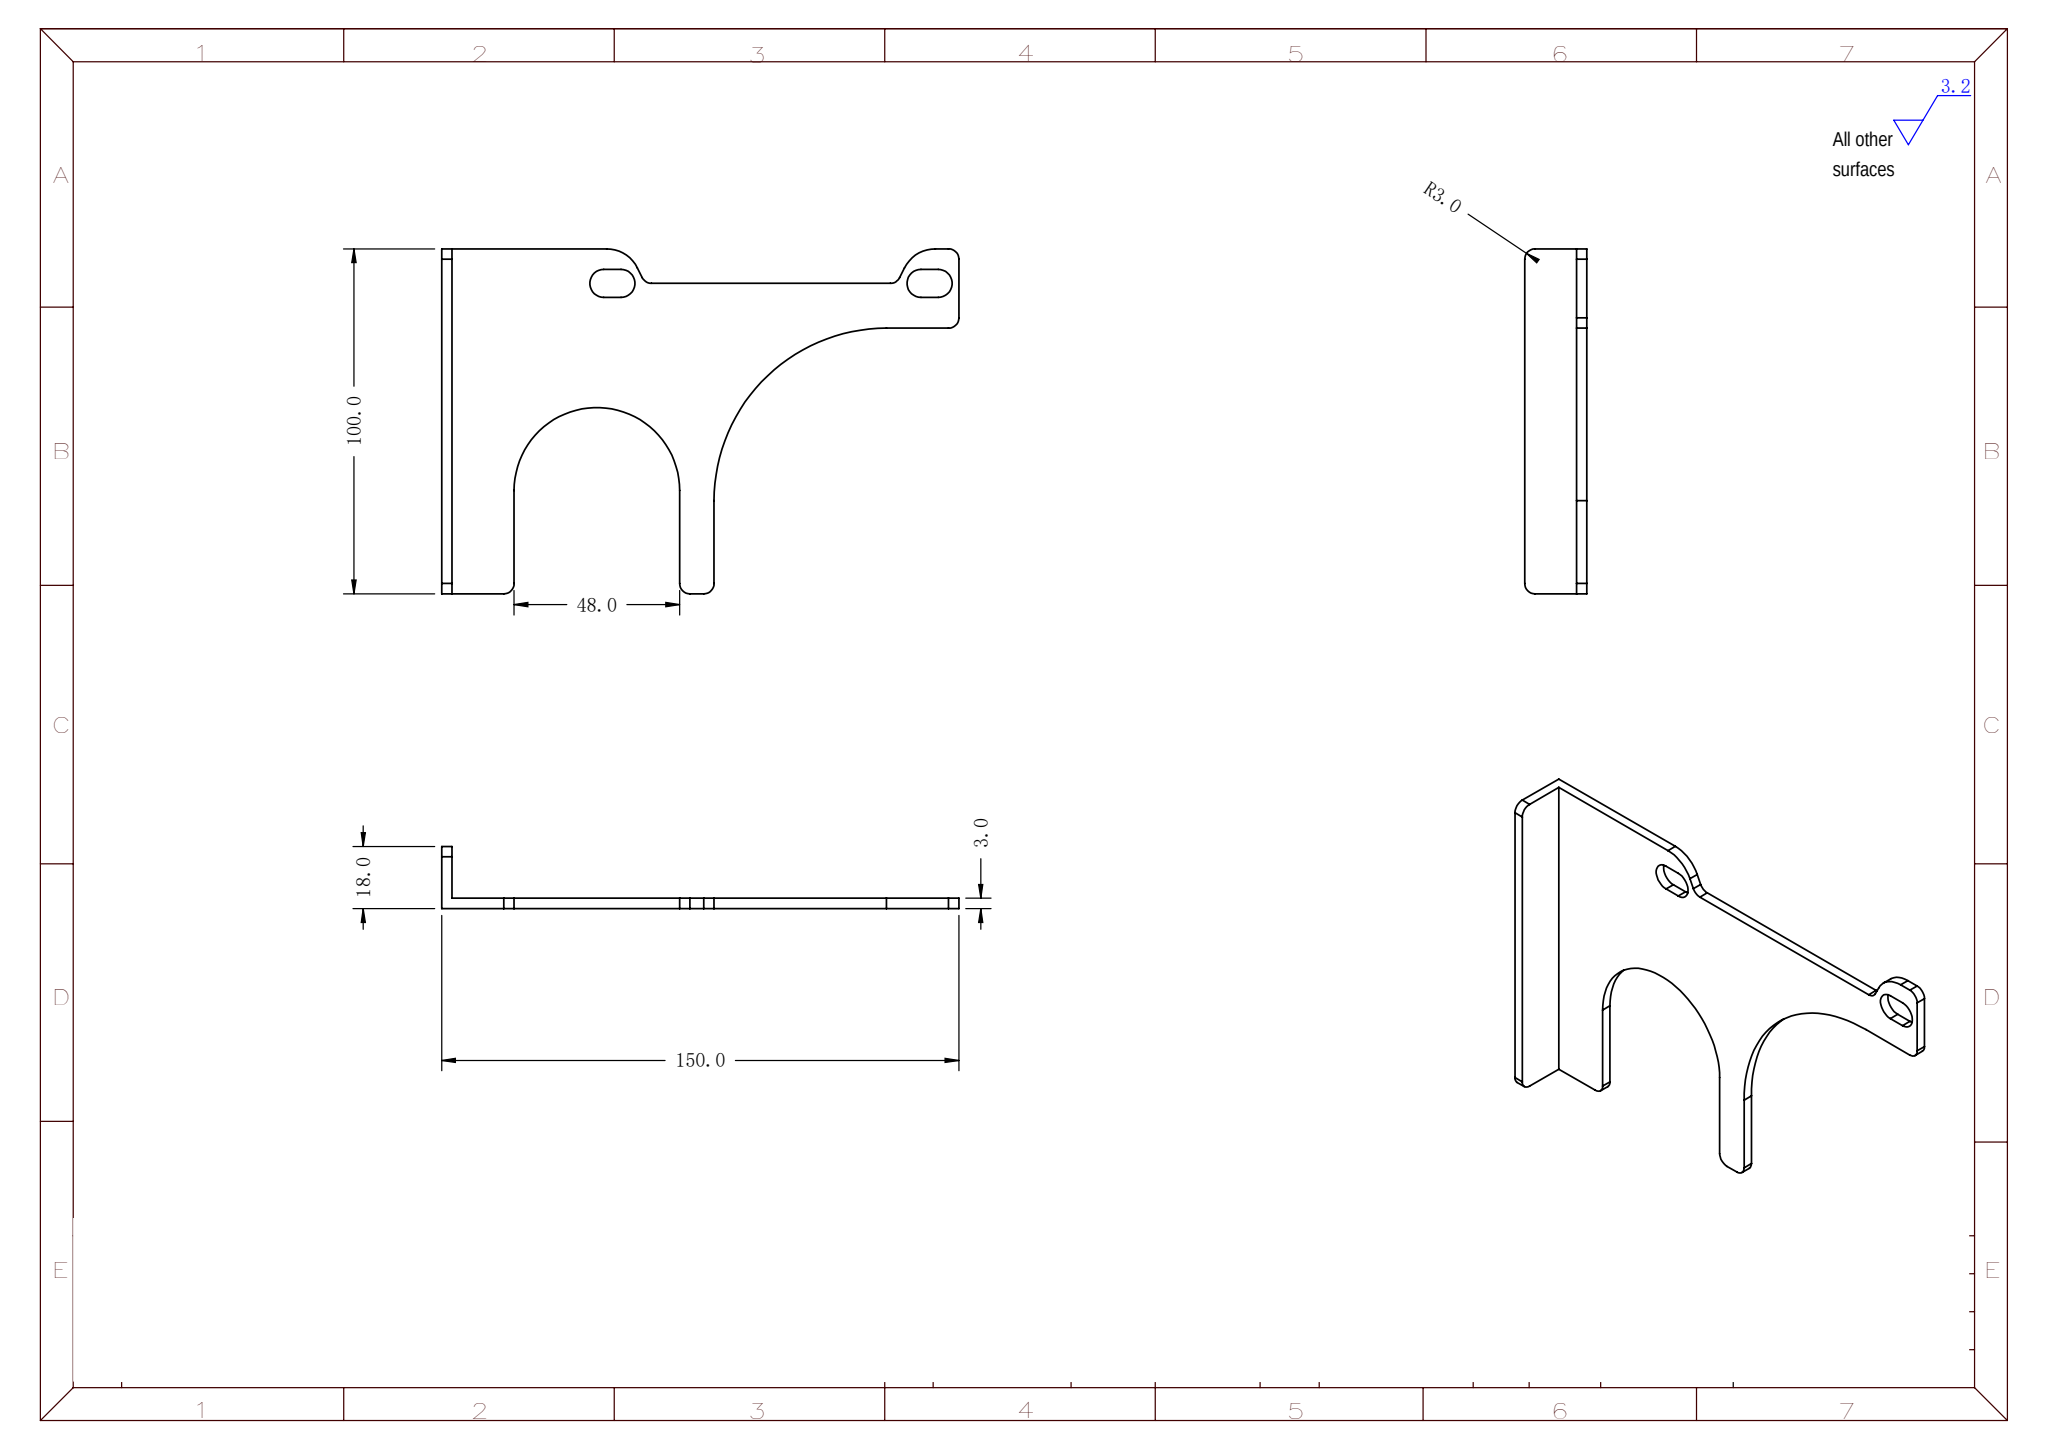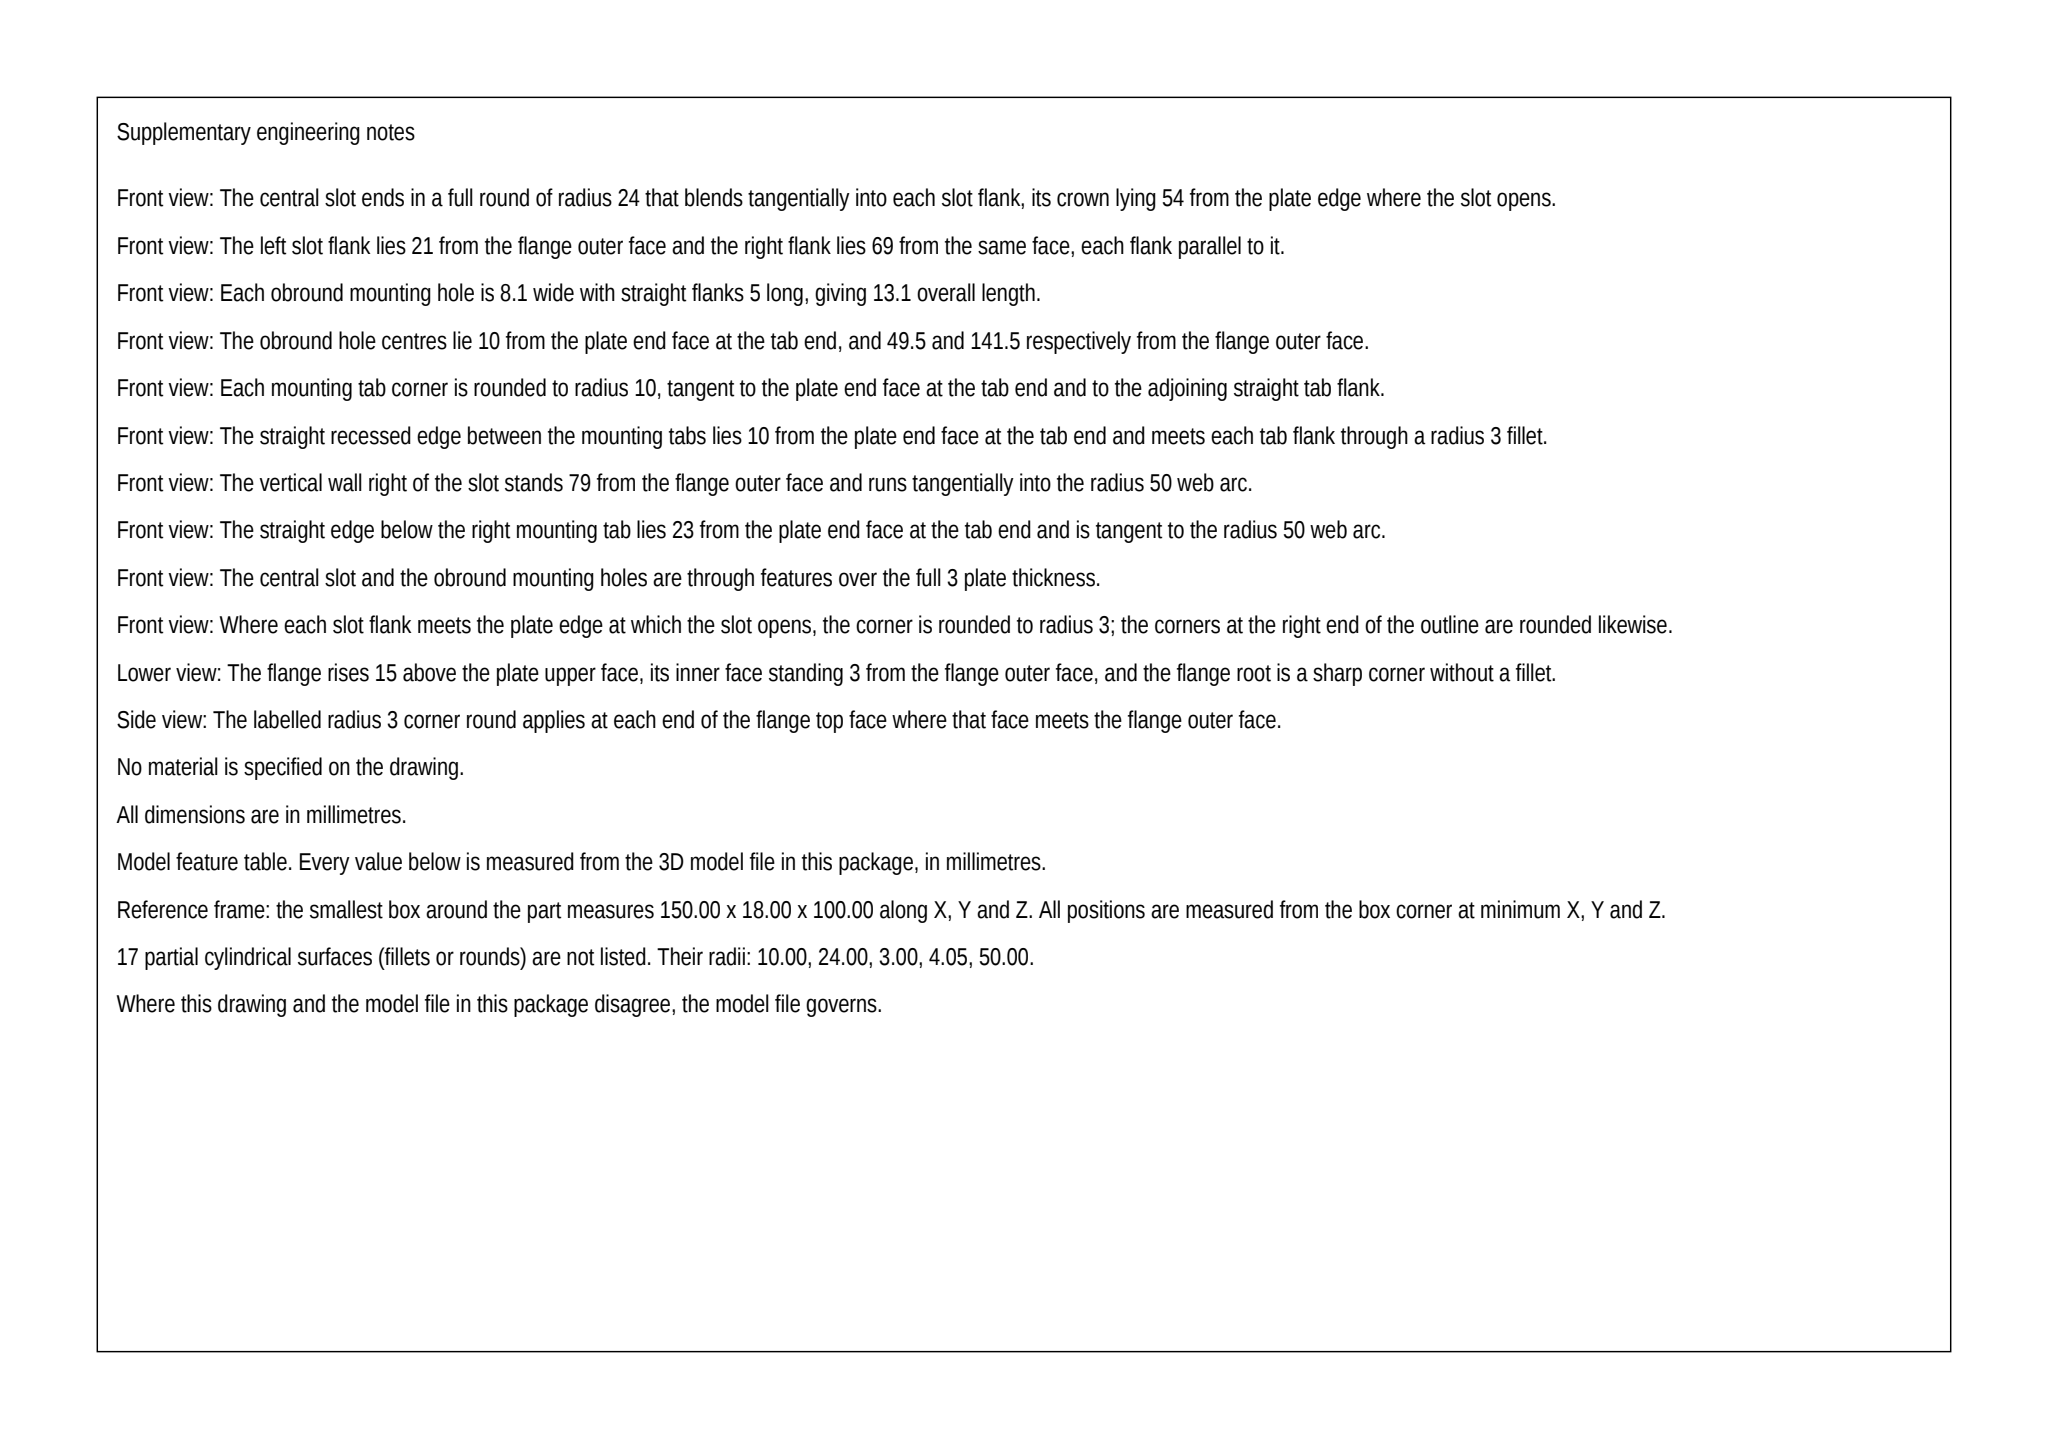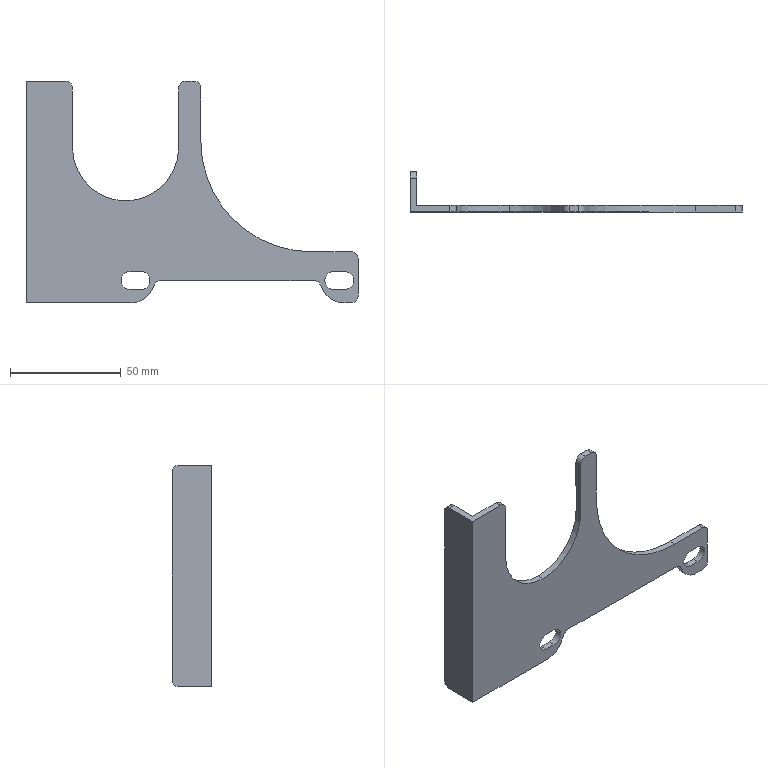Part | SolidWorks | mm | 1 solid | 39 faces | box 150 x 18 x 100 mm | volume 24706 mm3 | plane 21 | cylinder 18 | commonest cylinder face diameters 6 x9 8.1 x4 48 x2 20 x2 100 x1
Drawing notes:
ALL DIMENSIONS IN MILLIMETRES (mm). | from the solid: STEP bbox_xyz [150.0,18.0,100.0] given in mm
2X SLOT 8.1 WIDE X 13.1 LONG THRU (3.0 PLATE); SLOT CENTRES AT X=49.5 AND X=141.5 FROM LEFT EDGE (X0), BOTH 10.0 BELOW TOP EDGE. CENTRE-TO-CENTRE 92.0. | from the solid: cylinders dia 8.1 axis y at x=47.0 & 52.0 and x=139.0 & 144.0, all z=10.0, length 3.0
2X R10.0 LUG OUTER ARC: ARC CENTRES AT X=47.82 AND X=143.18 FROM LEFT EDGE (X0), 10.0 BELOW TOP EDGE (NOT CONCENTRIC WITH SLOTS). | from the solid: cylinders dia 20.0 axis y at [47.82,null,10.0] and [143.18,null,10.0]
ARCH CUTOUT R24.0 (48.0 WIDE) CENTRE AT X=45.0 FROM LEFT EDGE, 70.0 BELOW TOP EDGE; CUT STRAIGHT SIDES AT X=21.0 AND X=69.0. | from the solid: cylinder dia 48.0 axis y at [45.0,null,70.0]; x planes at 21.0 and 69.0
R50.0 UNDERSIDE FILLET, ARC CENTRE AT X=129.0 FROM LEFT EDGE, 73.0 BELOW TOP EDGE. | from the solid: cylinder dia 100.0 axis y at [129.0,null,73.0]
VERTICAL CUT EDGE AT X=79.0 FROM LEFT EDGE (X0). | from the solid: x plane at offset 79.0
TOP ARM UNDERSIDE FACE 10.0 BELOW TOP EDGE; SHOULDER FACE 23.0 BELOW TOP EDGE (=77.0 ABOVE BOTTOM EDGE). | from the solid: z planes at offsets 10.0 and 23.0 with overall z=100.0
R3.0 TYP AT ALL CORNERS AND EDGE BREAKS. | from the solid: cylinders dia 6.0 (R3.0) at x=18.0/72.0/76.0/147.0 and z=3.0/7.0/20.0/97.0
UPRIGHT FLANGE AT LEFT END: 18.0 HIGH, 3.0 THICK, OUTER FACE AT X=0, INNER FACE AT X=3.0. | from the solid: bbox y=18.0; x planes at 0.0 and 3.0; y planes at 0.0, 3.0, 18.0
ALL DIMENSIONS IN MILLIMETRES. | from the solid: STEP bbox_xyz [150.0, 18.0, 100.0] given in mm
2X 8.1 X 13.1 SLOT THRU 3.0 PLATE: slot centres 49.5 and 141.5 from left (plate) edge, 92.0 apart, both on a common centreline 10.0 from the top edge. | from the solid: cylinders dia 8.1 axis y at x=47.0 & 52.0 and x=139.0 & 144.0, all at z=10.0 (slot ends; 13.1 overall length, centres 49.5 / 141.5)
2X R10.0 OUTER LUG RADII: arc centres 47.82 and 143.18 from left edge, 10.0 from top edge (not concentric with the slots). | from the solid: cylinders dia 20.0 axis y at x=47.82, z=10.0 and x=143.18, z=10.0
R3.0 TYP ALL CORNER FILLETS (e.g. outer corner 147.0 from left edge, 20.0 from top edge). | from the solid: cylinders dia 6.0 (R3.0) axis y at x=18.0/72.0/76.0 z=97.0, x=60.85/130.15 z=7.0, x=147.0 z=3.0 and z=20.0
ARCH CUT-OUT 48.0 WIDE: left side 21.0 from left edge; apex 54.0 above the bottom edge (R24.0 arch, centre 45.0 from left edge). | from the solid: plane x=21.0 and x=69.0; cylinder dia 48.0 axis y at x=45.0, z=70.0 (apex 46.0 from top = 54.0 from bottom)
VERTICAL EDGE RIGHT OF ARCH: 79.0 from left edge, running up to 77.0 above the bottom edge where the R50.0 underside begins. | from the solid: plane x=79.0; plane z=23.0 (100.0 - 23.0 = 77.0 from bottom)
R50.0 CONCAVE ARM UNDERSIDE: arc centre 129.0 from left edge, 27.0 above the bottom edge. | from the solid: cylinder dia 100.0 axis y at x=129.0, z=73.0 (100.0 - 73.0 = 27.0 from bottom)
build123d program:
from build123d import *

# Parameters (mm, degrees)
BOSS_EXTRUDE1_DEPTH = 1.5
FILLET1_R           = 10
SKETCH2_W           = 3
SKETCH2_H           = 100
BOSS_EXTRUDE2_DEPTH = 15
FILLET2_R           = 3
FILLET3_R           = 50


with BuildPart() as part:
    # Sketch1 → Boss-Extrude1 (new, symmetric)
    with BuildSketch(Plane(origin=(0, 0, 0), x_dir=(1, 0, 0), z_dir=(0, 1, 0))):
        with BuildLine():
            Line((0, 0), (0, 100))
            Line((0, 100), (54, 100))
            Line((54, 100), (59, 90))
            Line((59, 90), (132, 90))
            Line((132, 90), (137, 100))
            Line((137, 100), (150, 100))
            Line((150, 100), (150, 77))
            Line((150, 77), (79, 77))
            Line((79, 77), (79, 0))
            Line((79, 0), (69, 0))
            Line((69, 0), (69, 30))
            ThreePointArc((69, 30), (45, 54), (21, 30))
            Line((21, 30), (21, 0))
            Line((21, 0), (0, 0))
        make_face()
        with BuildLine():
            Line((139, 94.05), (144, 94.05))
            ThreePointArc((144, 94.05), (148.05, 90), (144, 85.95))
            Line((144, 85.95), (139, 85.95))
            ThreePointArc((139, 85.95), (134.95, 90), (139, 94.05))
        make_face(mode=Mode.SUBTRACT)
        with BuildLine():
            Line((47, 94.05), (52, 94.05))
            ThreePointArc((52, 94.05), (56.05, 90), (52, 85.95))
            Line((52, 85.95), (47, 85.95))
            ThreePointArc((47, 85.95), (42.95, 90), (47, 94.05))
        make_face(mode=Mode.SUBTRACT)
    extrude(amount=BOSS_EXTRUDE1_DEPTH, both=True)

    # Fillet1
    fillet1_edges = [part.edges().sort_by_distance(p)[0] for p in [
        (54, 0, -100),
        (137, 0, -100),
    ]]
    fillet(fillet1_edges, radius=FILLET1_R)

    # Sketch2 → Boss-Extrude2 (add)
    with BuildSketch(Plane(origin=(0, 1.5, 0), x_dir=(1, 0, 0), z_dir=(0, 1, 0))):
        with Locations((1.5, 50)):
            Rectangle(SKETCH2_W, SKETCH2_H)
    extrude(amount=BOSS_EXTRUDE2_DEPTH)

    # Fillet2
    fillet2_edges = [part.edges().sort_by_distance(p)[0] for p in [
        (59, 0, -90),
        (132, 0, -90),
        (150, 0, -100),
        (150, 0, -77),
        (79, 0, 0),
        (69, 0, 0),
        (21, 0, 0),
        (1.5, 16.5, 0),
        (1.5, 16.5, -100),
    ]]
    fillet(fillet2_edges, radius=FILLET2_R)

    # Fillet3
    fillet3_edges = [part.edges().sort_by_distance(p)[0] for p in [
        (79, 0, -77),
    ]]
    fillet(fillet3_edges, radius=FILLET3_R)


solid = part.part